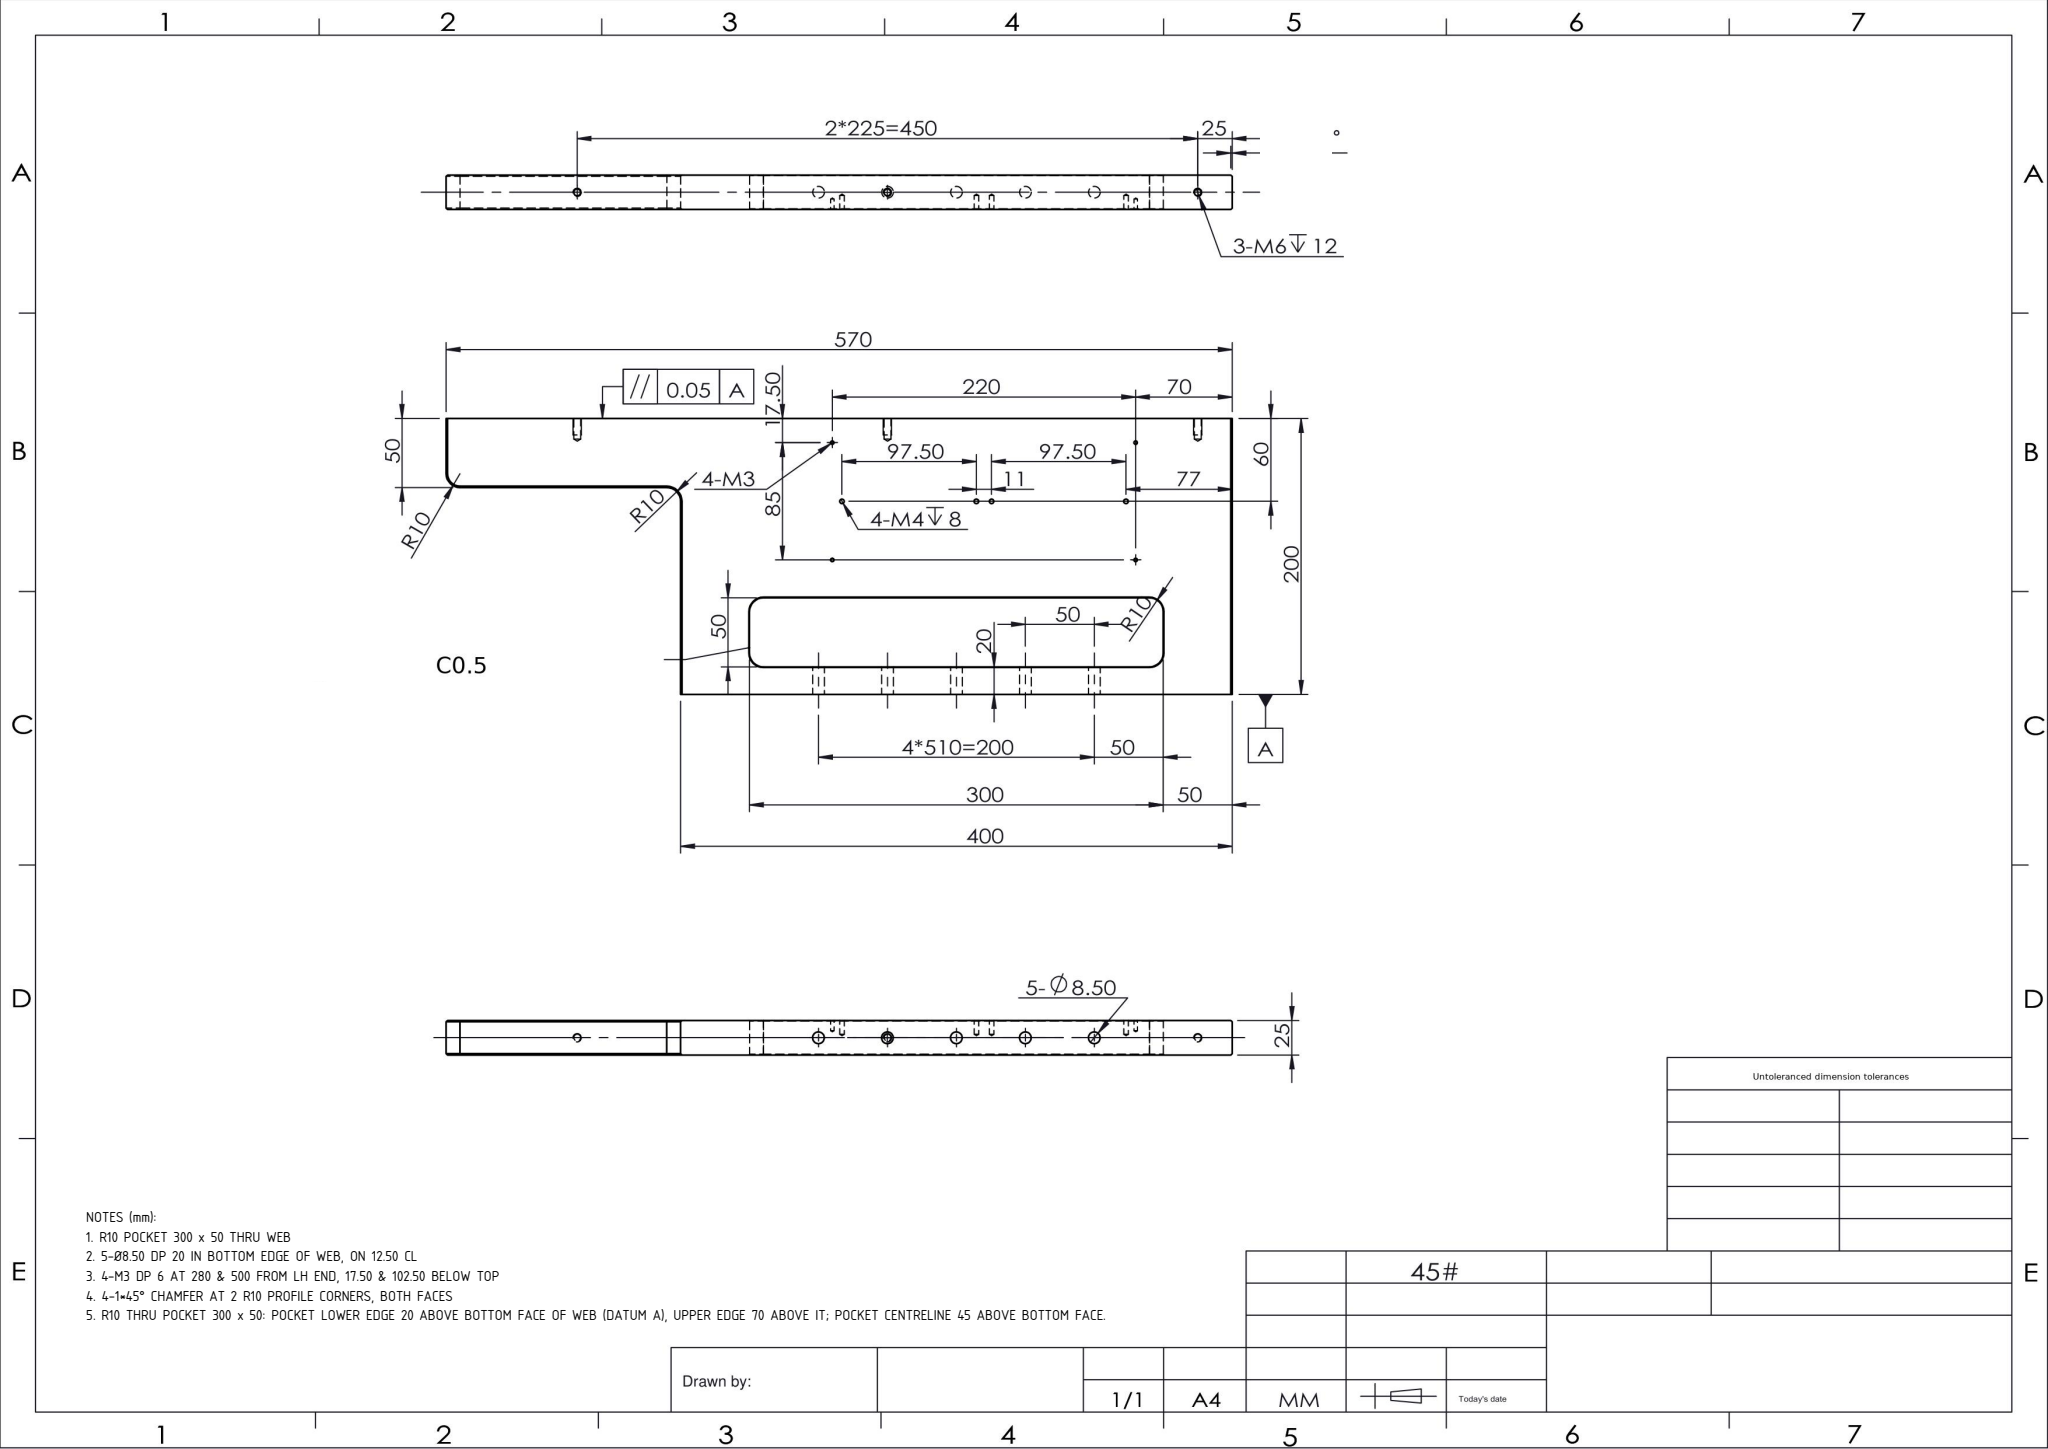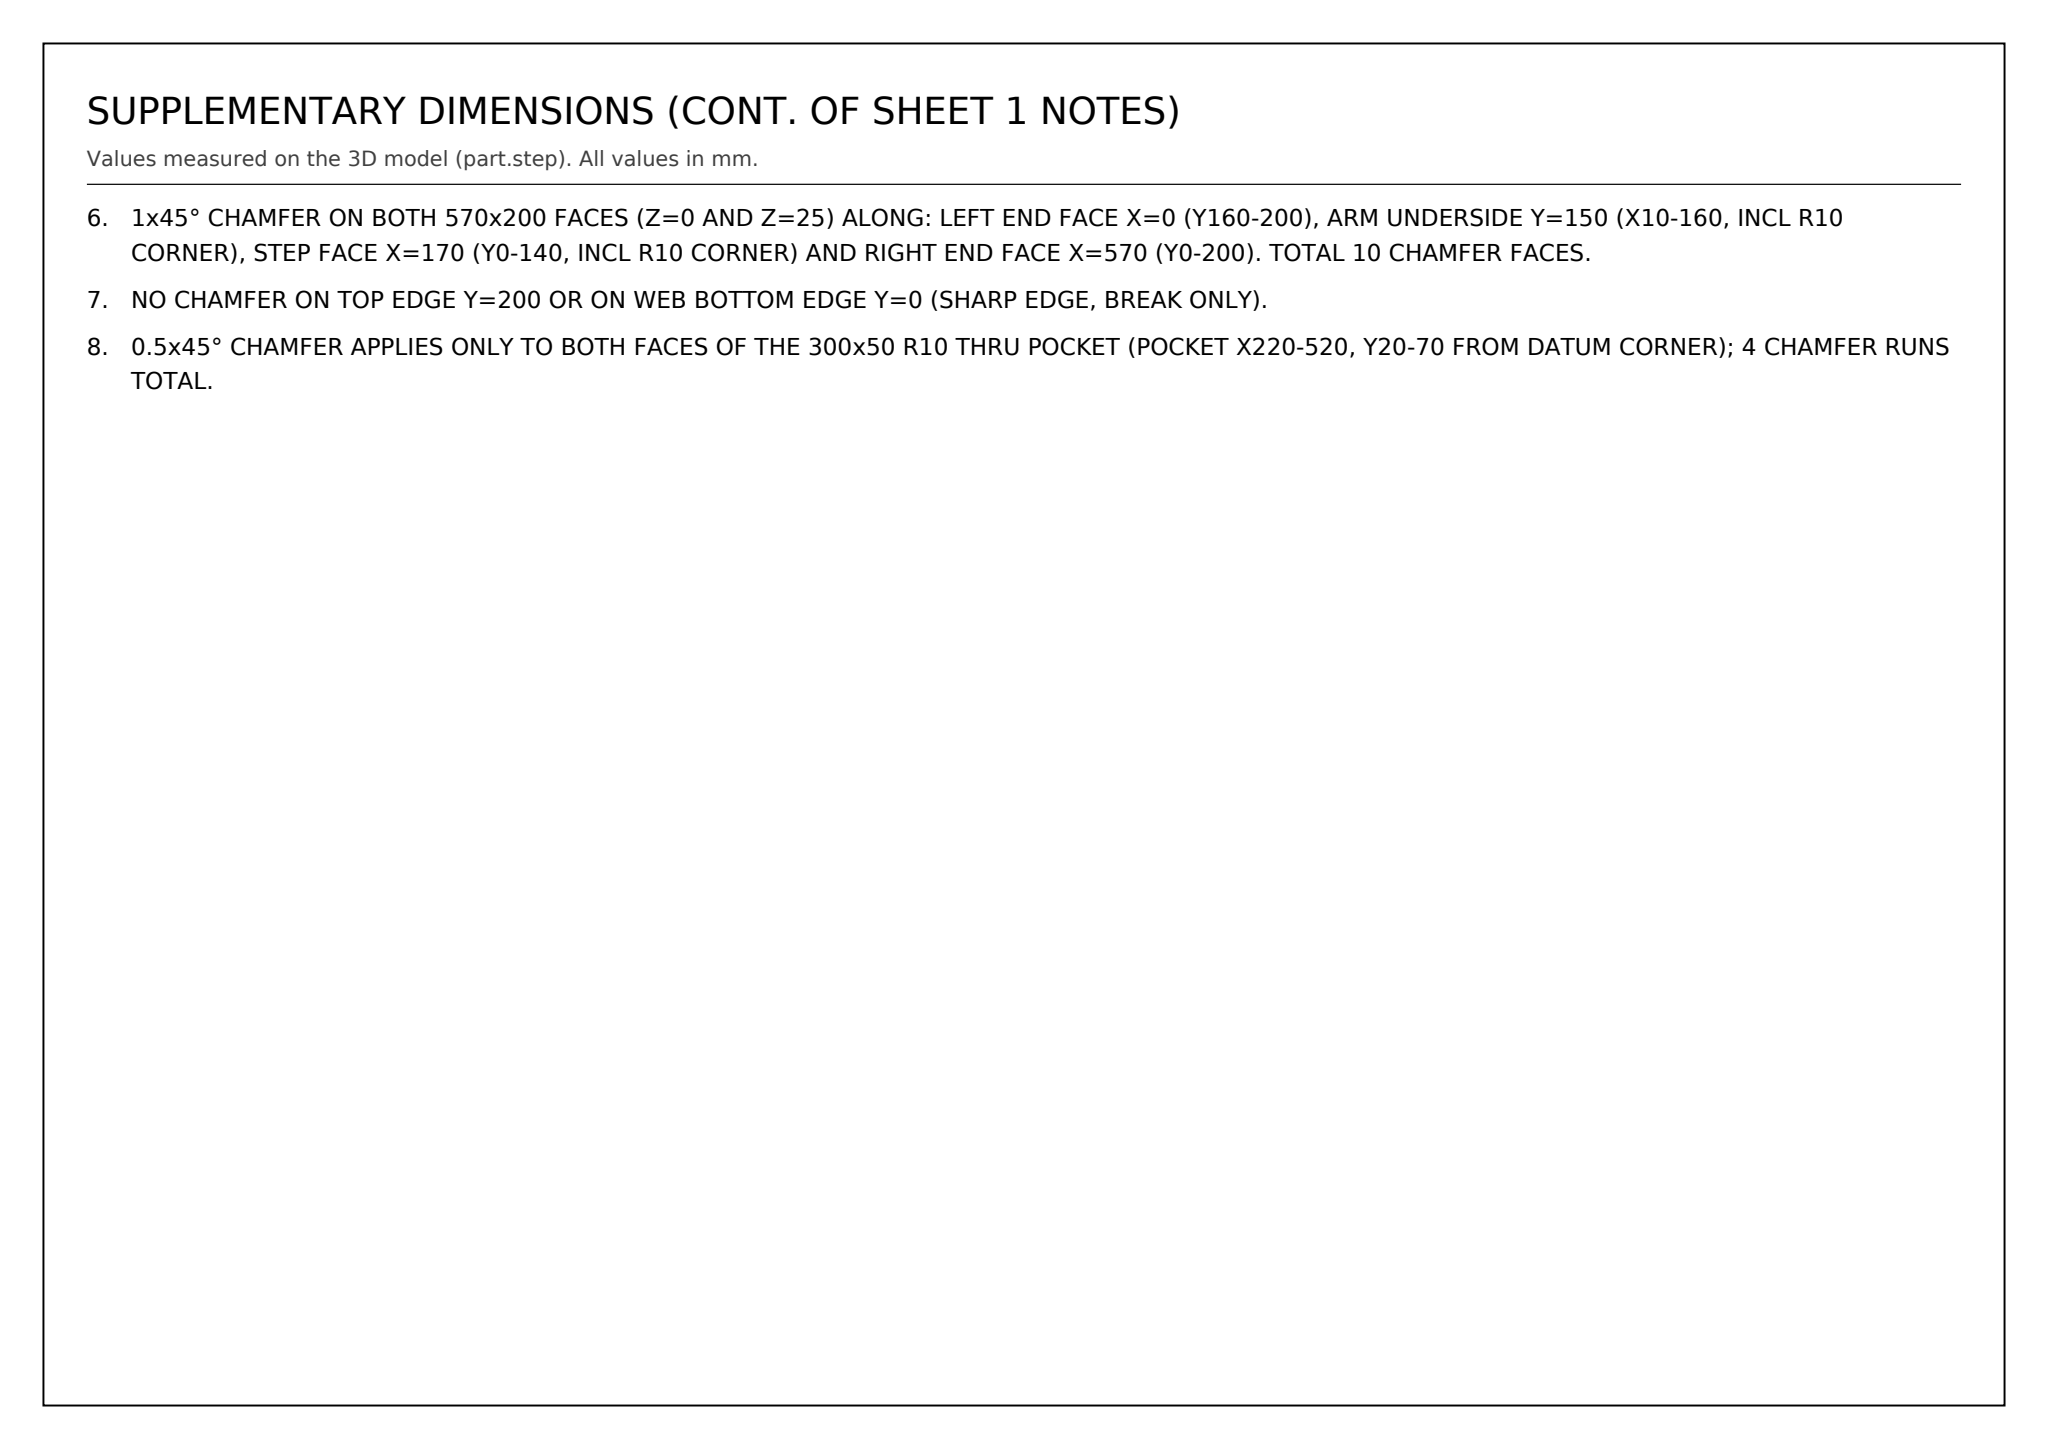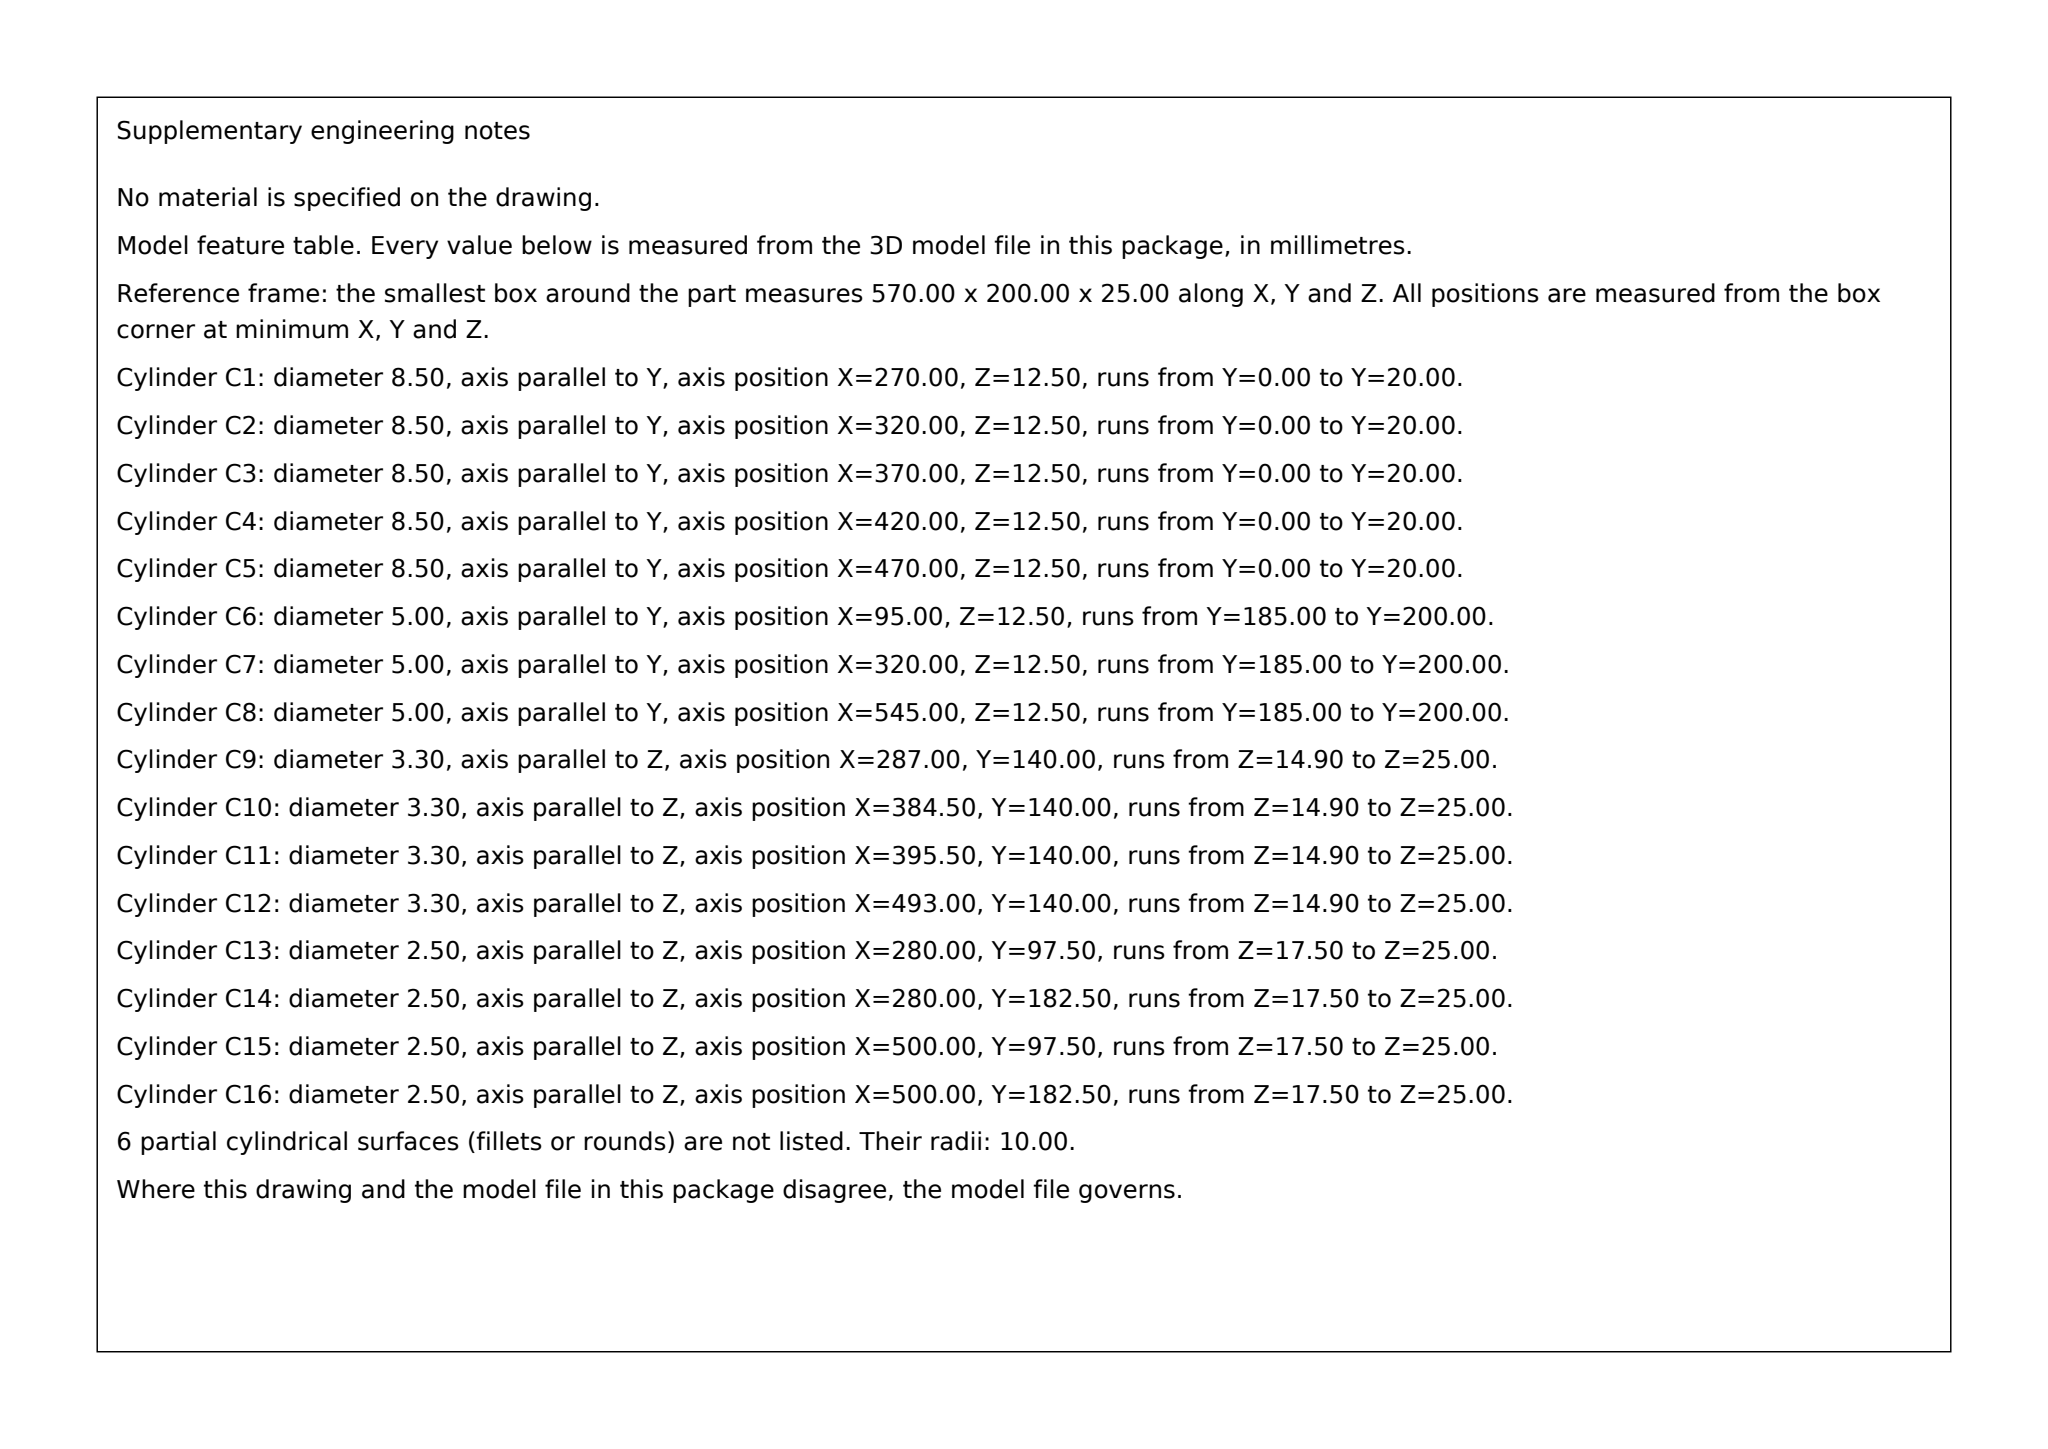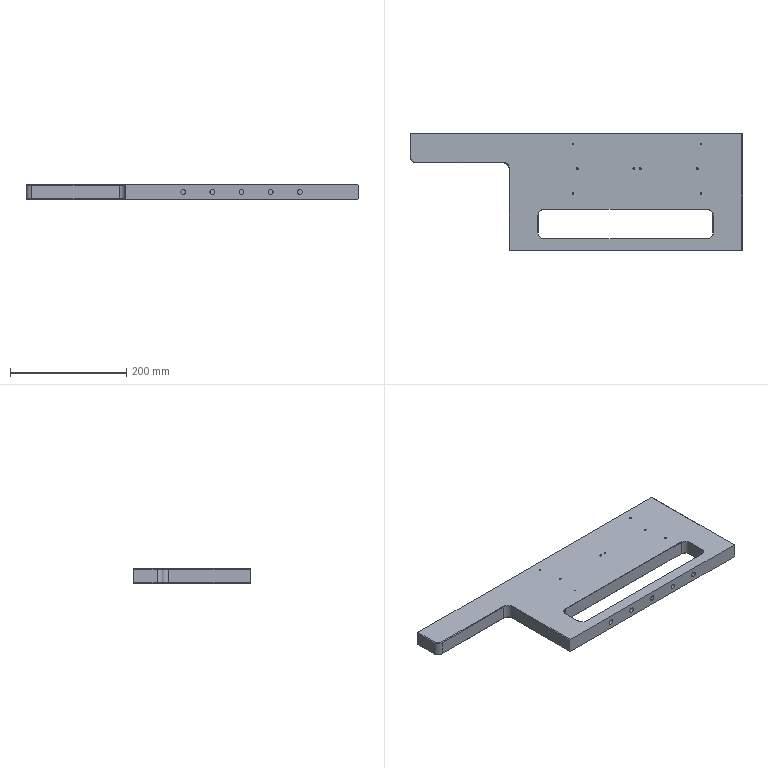Part | SolidWorks | mm | 1 solid | 100 faces | box 570 x 200 x 25 mm | volume 1831817 mm3 | cylinder 38 | cone 34 | plane 28 | commonest cylinder face diameters 8.5 x10 3.3 x8 2.5 x8 5 x6 20 x6
Drawing notes:
R10 POCKET 300 x 50 THRU WEB | from the solid: Pocket walls x=220/520, y=20/70, R10 corners at (230,30),(230,60),(510,30),(510,60); only z planes 0 and 25, no floor
5-Ø8.50 DP 20 IN BOTTOM EDGE OF WEB, ON 12.50 CL | from the solid: Ø8.5 y-axis blind holes at x=270/320/370/420/470, z=12.5, depth 20 from y=0 face
4-M3 DP 6 AT 280 & 500 FROM LH END, 17.50 & 102.50 BELOW TOP | from the solid: Ø2.5 z-axis tap drills len 7.5 at (280,97.5),(280,182.5),(500,97.5),(500,182.5) in 570x200 bbox
4-1*45° CHAMFER AT 2 R10 PROFILE CORNERS, BOTH FACES | from the solid: R10 corners Ø20 at (10,160) & (160,140) len 23 = 25-2x1; 90° cones Ø22 x2, Ø18 x2
R10 THRU POCKET 300 x 50: POCKET LOWER EDGE 20 ABOVE BOTTOM FACE OF WEB (DATUM A), UPPER EDGE 70 ABOVE IT; POCKET CENTRELINE 45 ABOVE BOTTOM FACE. | from the solid: axis_planes normal y at offset 20.0 (x 230-510, z 0.5-24.5) and offset 70.0 (x 230-510), with R10 corner arcs centred at y=30 and y=60
1x45° CHAMFER ON BOTH 570x200 FACES (Z=0 AND Z=25) ALONG: LEFT END FACE X=0 (Y160-200), ARM UNDERSIDE Y=150 (X10-160, INCL R10 CORNER), STEP FACE X=170 (Y0-140, INCL R10 CORNER) AND RIGHT END FACE X=570 (Y0-200). TOTAL 10 CHAMFER FACES. | from the solid: inclined_planes 45° of size 1.0 at bbox_from [0,160,0]/[0,160,24], [170,0,0]/[170,0,24], [569,0,0]/[569,0,24], [10,150,0]/[10,150,24]
NO CHAMFER ON TOP EDGE Y=200 OR ON WEB BOTTOM EDGE Y=0 (SHARP EDGE, BREAK ONLY). | from the solid: planes y=200 and y=0 have full z extent 0.0-25.0; no 45° inclined planes at y=0 or y=200
0.5x45° CHAMFER APPLIES ONLY TO BOTH FACES OF THE 300x50 R10 THRU POCKET (POCKET X220-520, Y20-70 FROM DATUM CORNER); 4 CHAMFER RUNS TOTAL. | from the solid: inclined_planes 45° of size 0.5 at bbox_from [219.5,30,0]/[219.5,30,24.5], [520,30,0]/[520,30,24.5], [230,19.5,0]/[230,19.5,24.5], [230,70,0]/[230,70,24.5]; pocket walls x=220/x=520 and y=20/y=70 run z 0.5-24.5
build123d program:
from build123d import *

# Parameters (mm, degrees)
SKETCH1_W             = 400
SKETCH1_H             = 200
BOSS_EXTRUDE1_DEPTH   = 25
SKETCH2_W             = 170
SKETCH2_H             = 50
BOSS_EXTRUDE2_DEPTH   = 25
FILLET1_R             = 10
SKETCH3_W             = 300
SKETCH3_H             = 50
CUT_EXTRUDE1_DEPTH    = 448.912
FILLET2_R             = 10
FILLET3_R             = 10
LPATTERN1_COUNT       = 3
LPATTERN1_PITCH       = 225
SKETCH6_R             = 4.25
CUT_EXTRUDE2_DEPTH    = 50
LPATTERN2_COUNT       = 5
LPATTERN2_PITCH       = 50
CHAMFER1_SIZE         = 1
CHAMFER2_SIZE         = 0.5
M3_TAPPED_HOLE1_D     = 2.5
M3_TAPPED_HOLE1_DEPTH = 7.5
M3_TAPPED_HOLE1_TIP   = 0.7511
M4_TAPPED_HOLE1_D     = 3.3
M4_TAPPED_HOLE1_DEPTH = 10.1
M4_TAPPED_HOLE1_TIP   = 0.9914


with BuildPart() as part:
    # Sketch1 → Boss-Extrude1 (new body)
    with BuildSketch(Plane.XY):
        with Locations((200, 100)):
            Rectangle(SKETCH1_W, SKETCH1_H)
    extrude(amount=BOSS_EXTRUDE1_DEPTH)

    # Sketch2 → Boss-Extrude2 (add)
    with BuildSketch(Plane.XY.offset(25)):
        with Locations((-85, 175)):
            Rectangle(SKETCH2_W, SKETCH2_H)
    extrude(amount=-BOSS_EXTRUDE2_DEPTH)

    # Fillet1
    fillet1_edges = [part.edges().sort_by_distance(p)[0] for p in [
        (0, 150, 12.5),
    ]]
    fillet(fillet1_edges, radius=FILLET1_R)

    # Sketch3 → Cut-Extrude1 (cut, through all)
    with BuildSketch(Plane.XY.offset(25)):
        with Locations((200, 45)):
            Rectangle(SKETCH3_W, SKETCH3_H)
    extrude(amount=-CUT_EXTRUDE1_DEPTH, mode=Mode.SUBTRACT)

    # Fillet2
    fillet2_edges = [part.edges().sort_by_distance(p)[0] for p in [
        (50, 20, 12.5),
        (50, 70, 12.5),
        (350, 70, 12.5),
        (350, 20, 12.5),
    ]]
    fillet(fillet2_edges, radius=FILLET2_R)

    # Fillet3
    fillet3_edges = [part.edges().sort_by_distance(p)[0] for p in [
        (-170, 150, 12.5),
    ]]
    fillet(fillet3_edges, radius=FILLET3_R)

    # Sketch4 → M6 Tapped Hole1 (revolve, cut)
    with BuildSketch(Plane(origin=(375, 200, 12.5), x_dir=(0, 0, 1), z_dir=(1, 0, 0))):
        Polygon((0, 0), (0, 16.502), (2.5, 15), (2.5, 0), align=None)
    m6_tapped_hole1 = revolve(axis=Axis((375, 206.35, 12.5), (0, -1, 0)), mode=Mode.SUBTRACT)

    # LPattern1: M6 Tapped Hole1 ×3
    with Locations(*[(-i * LPATTERN1_PITCH, 0, 0) for i in range(1, LPATTERN1_COUNT)]):
        add(m6_tapped_hole1, mode=Mode.SUBTRACT)

    # Sketch6 → Cut-Extrude2 (cut)
    with BuildSketch(Plane(origin=(0, 0, 0), x_dir=(-1, 0, 0), z_dir=(0, -1, 0))):
        with Locations(Location((-100, -12.5, 0), (0, 0, 90))):
            Circle(SKETCH6_R)
    cut_extrude2 = extrude(amount=-CUT_EXTRUDE2_DEPTH, mode=Mode.SUBTRACT)

    # LPattern2: Cut-Extrude2 ×5
    with Locations(*[(i * LPATTERN2_PITCH, 0, 0) for i in range(1, LPATTERN2_COUNT)]):
        add(cut_extrude2, mode=Mode.SUBTRACT)

    # Chamfer1
    chamfer1_edges = [part.edges().sort_by_distance(p)[0] for p in [
        (400, 100, 25),
        (-170, 180, 0),
        (-170, 180, 25),
        (0, 70, 0),
        (0, 70, 25),
        (-2.929, 147.071, 25),
        (-2.929, 147.071, 0),
        (400, 100, 0),
        (-85, 150, 25),
        (-167.071, 152.929, 25),
        (-85, 150, 0),
        (-167.071, 152.929, 0),
    ]]
    chamfer(chamfer1_edges, length=CHAMFER1_SIZE)

    # Chamfer2
    chamfer2_edges = [part.edges().sort_by_distance(p)[0] for p in [
        (50, 45, 25),
        (50, 45, 0),
        (200, 70, 25),
        (200, 70, 0),
        (350, 45, 25),
        (350, 45, 0),
        (200, 20, 25),
        (200, 20, 0),
        (52.929, 67.071, 25),
        (52.929, 67.071, 0),
        (347.071, 67.071, 25),
        (347.071, 67.071, 0),
        (347.071, 22.929, 25),
        (347.071, 22.929, 0),
        (52.929, 22.929, 25),
        (52.929, 22.929, 0),
    ]]
    chamfer(chamfer2_edges, length=CHAMFER2_SIZE)

    # M3 Tapped Hole1
    with Locations(Plane.XY.offset(25)):
        with Locations((110, 182.5), (330, 97.5), (330, 182.5), (110, 97.5)):
            Hole(M3_TAPPED_HOLE1_D / 2, depth=M3_TAPPED_HOLE1_DEPTH)
            with Locations((0, 0, -(M3_TAPPED_HOLE1_DEPTH + M3_TAPPED_HOLE1_TIP / 2))):  # 118° drill point
                Cone(0, M3_TAPPED_HOLE1_D / 2, M3_TAPPED_HOLE1_TIP, mode=Mode.SUBTRACT)

    # M4 Tapped Hole1
    with Locations(Plane.XY.offset(25)):
        with Locations((117, 140), (214.5, 140), (225.5, 140), (323, 140)):
            Hole(M4_TAPPED_HOLE1_D / 2, depth=M4_TAPPED_HOLE1_DEPTH)
            with Locations((0, 0, -(M4_TAPPED_HOLE1_DEPTH + M4_TAPPED_HOLE1_TIP / 2))):  # 118° drill point
                Cone(0, M4_TAPPED_HOLE1_D / 2, M4_TAPPED_HOLE1_TIP, mode=Mode.SUBTRACT)


solid = part.part